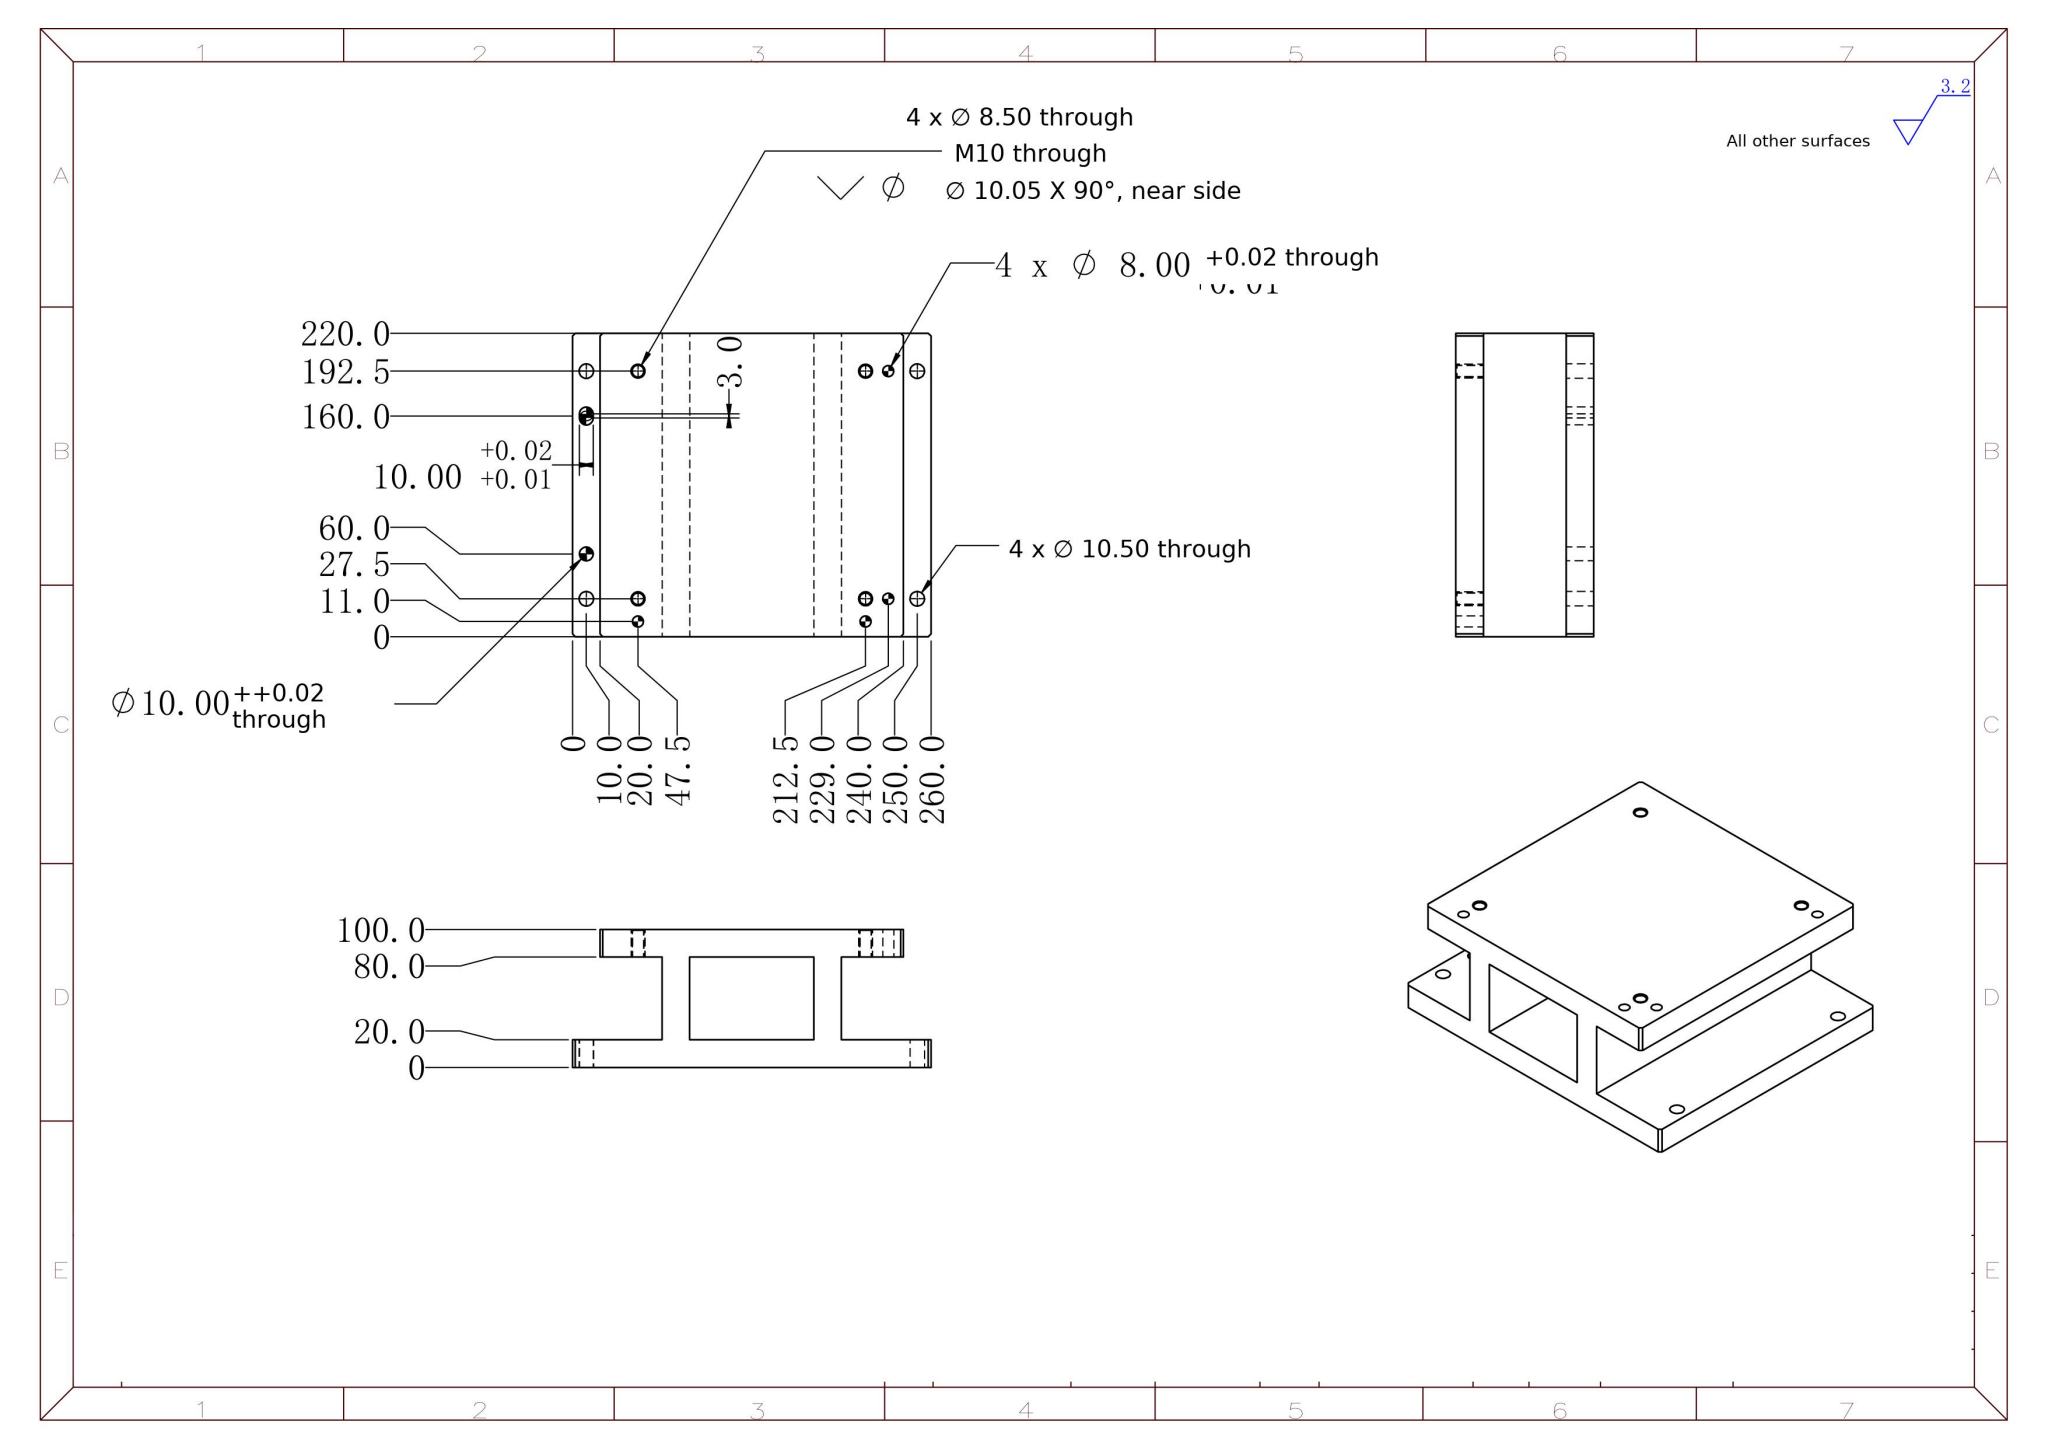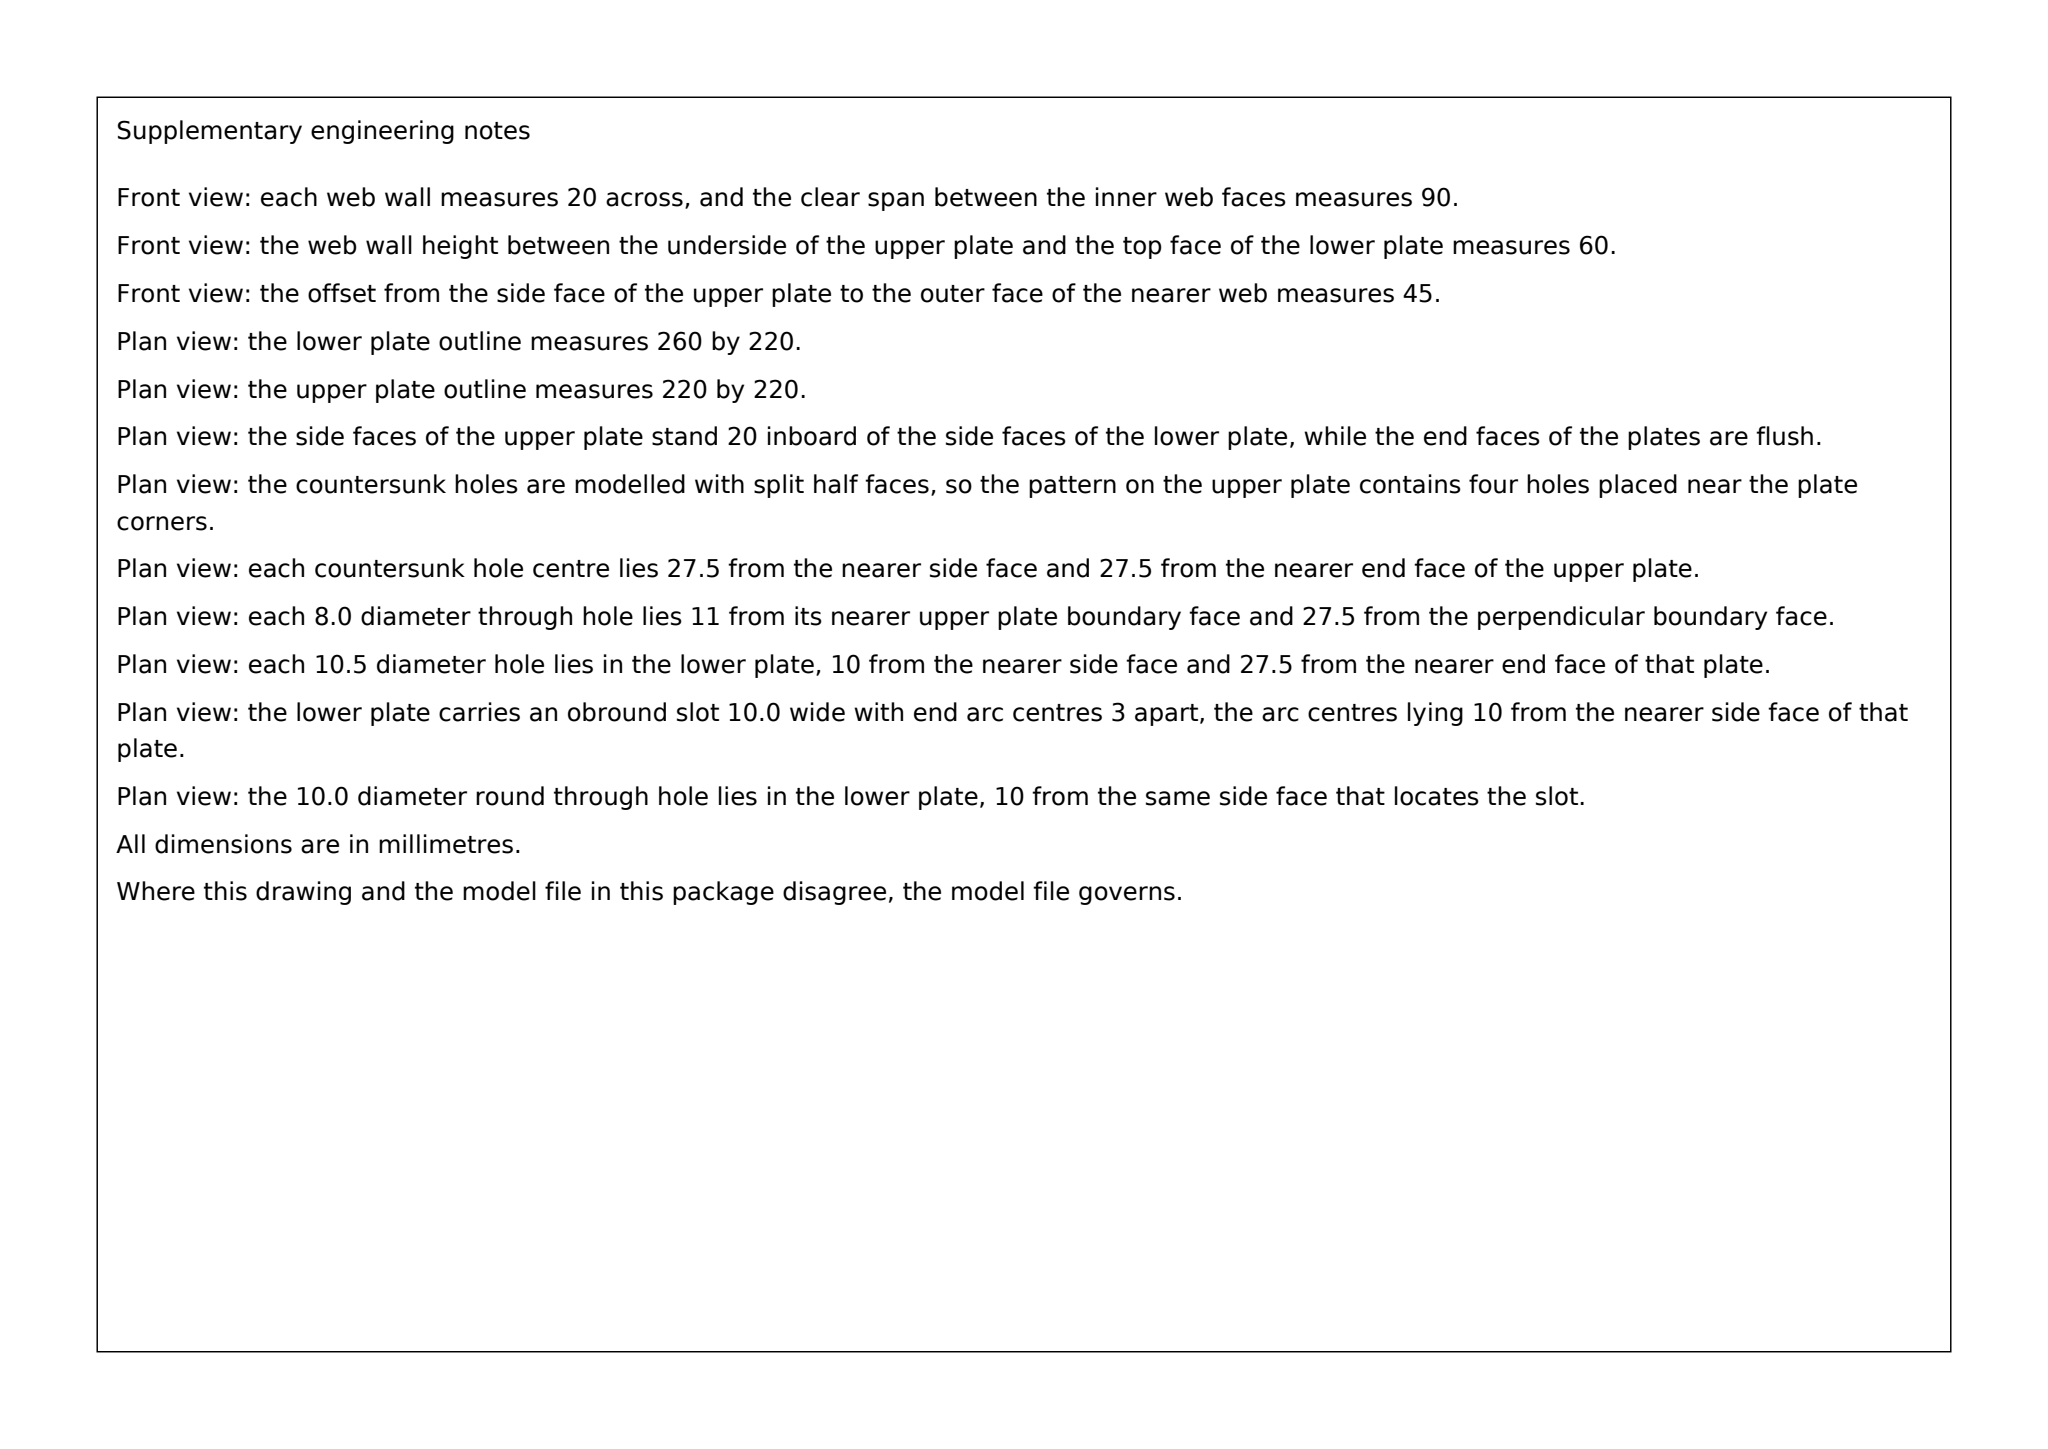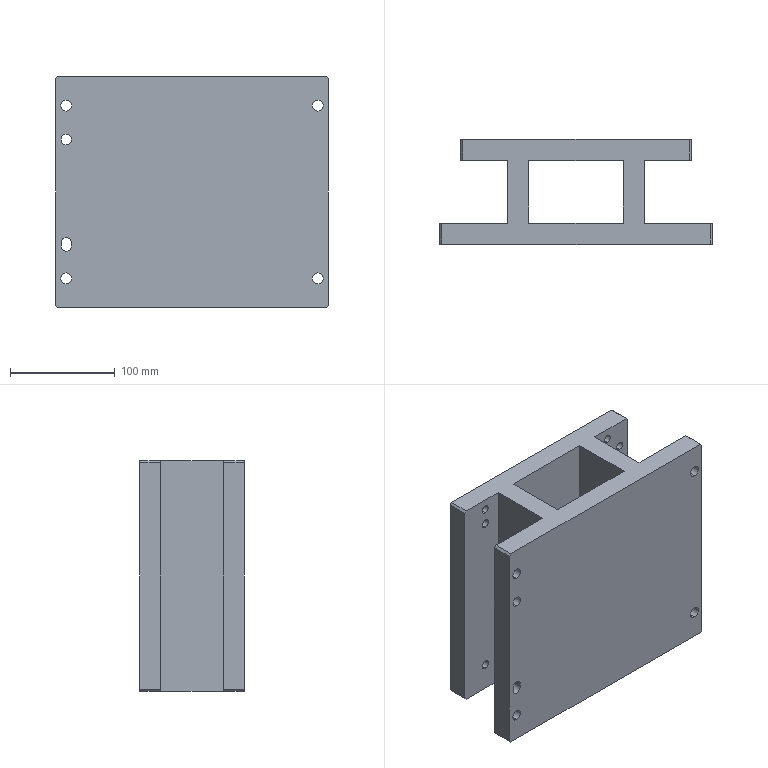Part | SolidWorks | mm | 1 solid | 65 faces | box 260 x 100 x 220 mm | volume 2620416 mm3 | cylinder 29 | plane 28 | cone 8 | commonest cylinder face diameters 10.5 x8 8 x8 8.5 x8 10 x5
Drawing notes:
2 X WEB: X=65-85 & X=175-195 FROM LH EDGE (SEE FRONT VIEW) | from the solid: axis_planes x at 65,85,175,195; bbox X=260 datum at x=0
WEB THK 20, TYP 2 PL | from the solid: x planes 65->85 and 175->195 = 20 each
CENTER OPENING 90 WIDE BETWEEN WEBS (X=85 TO 175) | from the solid: x planes 85 and 175, 175-85=90
ALL HOLES THRU EA FLANGE 20 THK, TOP & BOT, NOT THRU 100 | from the solid: all cylinders axis y, length 20 (8.5 dia 19.23 + CSK), count 2 each at same X,Z; y planes 0/20 and 80/100
FRONT VIEW: 2 x Ø8.00 +0.02/+0.01 AT Z=209.0 FROM 0 DATUM | from the solid: cyl dia 8.0 axis y at [47.5,null,209.0] and [212.5,null,209.0]; z datum 0 = bbox min, z-plane 0.0
build123d program:
from build123d import *

# Parameters (mm, degrees)
SKETCH3_W                     = 220
SKETCH3_H                     = 220
BOSS_EXTRUDE2_DEPTH           = 20
SKETCH4_W                     = 20
SKETCH4_H                     = 220
BOSS_EXTRUDE3_DEPTH           = 60
SKETCH5_W                     = 260
SKETCH5_H                     = 220
SKETCH5_R                     = 5
BOSS_EXTRUDE4_DEPTH           = 20
M10_TAPPED_HOLE1_D            = 8.5
M10_TAPPED_HOLE1_DEPTH        = 20
M10_TAPPED_HOLE1_CSINK_D      = 10.05
M10_TAPPED_HOLE1_CSINK_ANGLE  = 90
SIZE_MM_DOWEL_PIN_HOLE1_D     = 8
SIZE_MM_DOWEL_PIN_HOLE1_DEPTH = 20
M10_CLEARANCE_HOLE1_D         = 10.5
CHAMFER1_SIZE                 = 2


with BuildPart() as part:
    # Sketch3 → Boss-Extrude2 (new body)
    with BuildSketch(Plane(origin=(0, 0, 0), x_dir=(1, 0, 0), z_dir=(0, 1, 0))):
        Rectangle(SKETCH3_W, SKETCH3_H)
    extrude(amount=BOSS_EXTRUDE2_DEPTH)

    # Sketch4 → Boss-Extrude3 (add)
    with BuildSketch(Plane.XZ):
        with Locations((-55, 0)):
            Rectangle(SKETCH4_W, SKETCH4_H)
        with Locations((55, 0)):
            Rectangle(SKETCH4_W, SKETCH4_H)
    extrude(amount=BOSS_EXTRUDE3_DEPTH)

    # Sketch5 → Boss-Extrude4 (add)
    with BuildSketch(Plane.XZ.offset(60)):
        Rectangle(SKETCH5_W, SKETCH5_H)
        with Locations(Location((-120, 50, 0), (0, 0, 270))):
            Circle(SKETCH5_R, mode=Mode.SUBTRACT)
        with BuildLine():
            Line((-115, -48.5), (-115, -51.5))
            ThreePointArc((-115, -51.5), (-120, -56.5), (-125, -51.5))
            Line((-125, -51.5), (-125, -48.5))
            ThreePointArc((-125, -48.5), (-120, -43.5), (-115, -48.5))
        make_face(mode=Mode.SUBTRACT)
    extrude(amount=BOSS_EXTRUDE4_DEPTH)

    # M10 Tapped Hole1
    with Locations(Plane(origin=(0, 20, 0), x_dir=(1, 0, 0), z_dir=(0, 1, 0))):
        with Locations((-82.5, 82.5), (-82.5, -82.5), (82.5, 82.5), (82.5, -82.5)):
            CounterSinkHole(M10_TAPPED_HOLE1_D / 2, M10_TAPPED_HOLE1_CSINK_D / 2, depth=M10_TAPPED_HOLE1_DEPTH, counter_sink_angle=M10_TAPPED_HOLE1_CSINK_ANGLE)

    # Size mm Dowel Pin Hole1
    with Locations(Plane(origin=(0, 20, 0), x_dir=(1, 0, 0), z_dir=(0, 1, 0))):
        with Locations((-82.5, -99), (82.5, -99), (99, -82.5), (99, 82.5)):
            Hole(SIZE_MM_DOWEL_PIN_HOLE1_D / 2, depth=SIZE_MM_DOWEL_PIN_HOLE1_DEPTH)

    # M10 Clearance Hole1 (through all)
    with Locations(Plane(origin=(0, -60, 0), x_dir=(1, 0, 0), z_dir=(0, 1, 0))):
        with Locations((120, -82.5), (-120, -82.5), (120, 82.5), (-120, 82.5)):
            Hole(M10_CLEARANCE_HOLE1_D / 2)

    # Chamfer1
    chamfer1_edges = [part.edges().sort_by_distance(p)[0] for p in [
        (130, -70, -110),
        (130, -70, 110),
        (-130, -70, 110),
        (-130, -70, -110),
        (110, 10, 110),
        (-110, 10, 110),
        (-110, 10, -110),
        (110, 10, -110),
    ]]
    chamfer(chamfer1_edges, length=CHAMFER1_SIZE)


solid = part.part